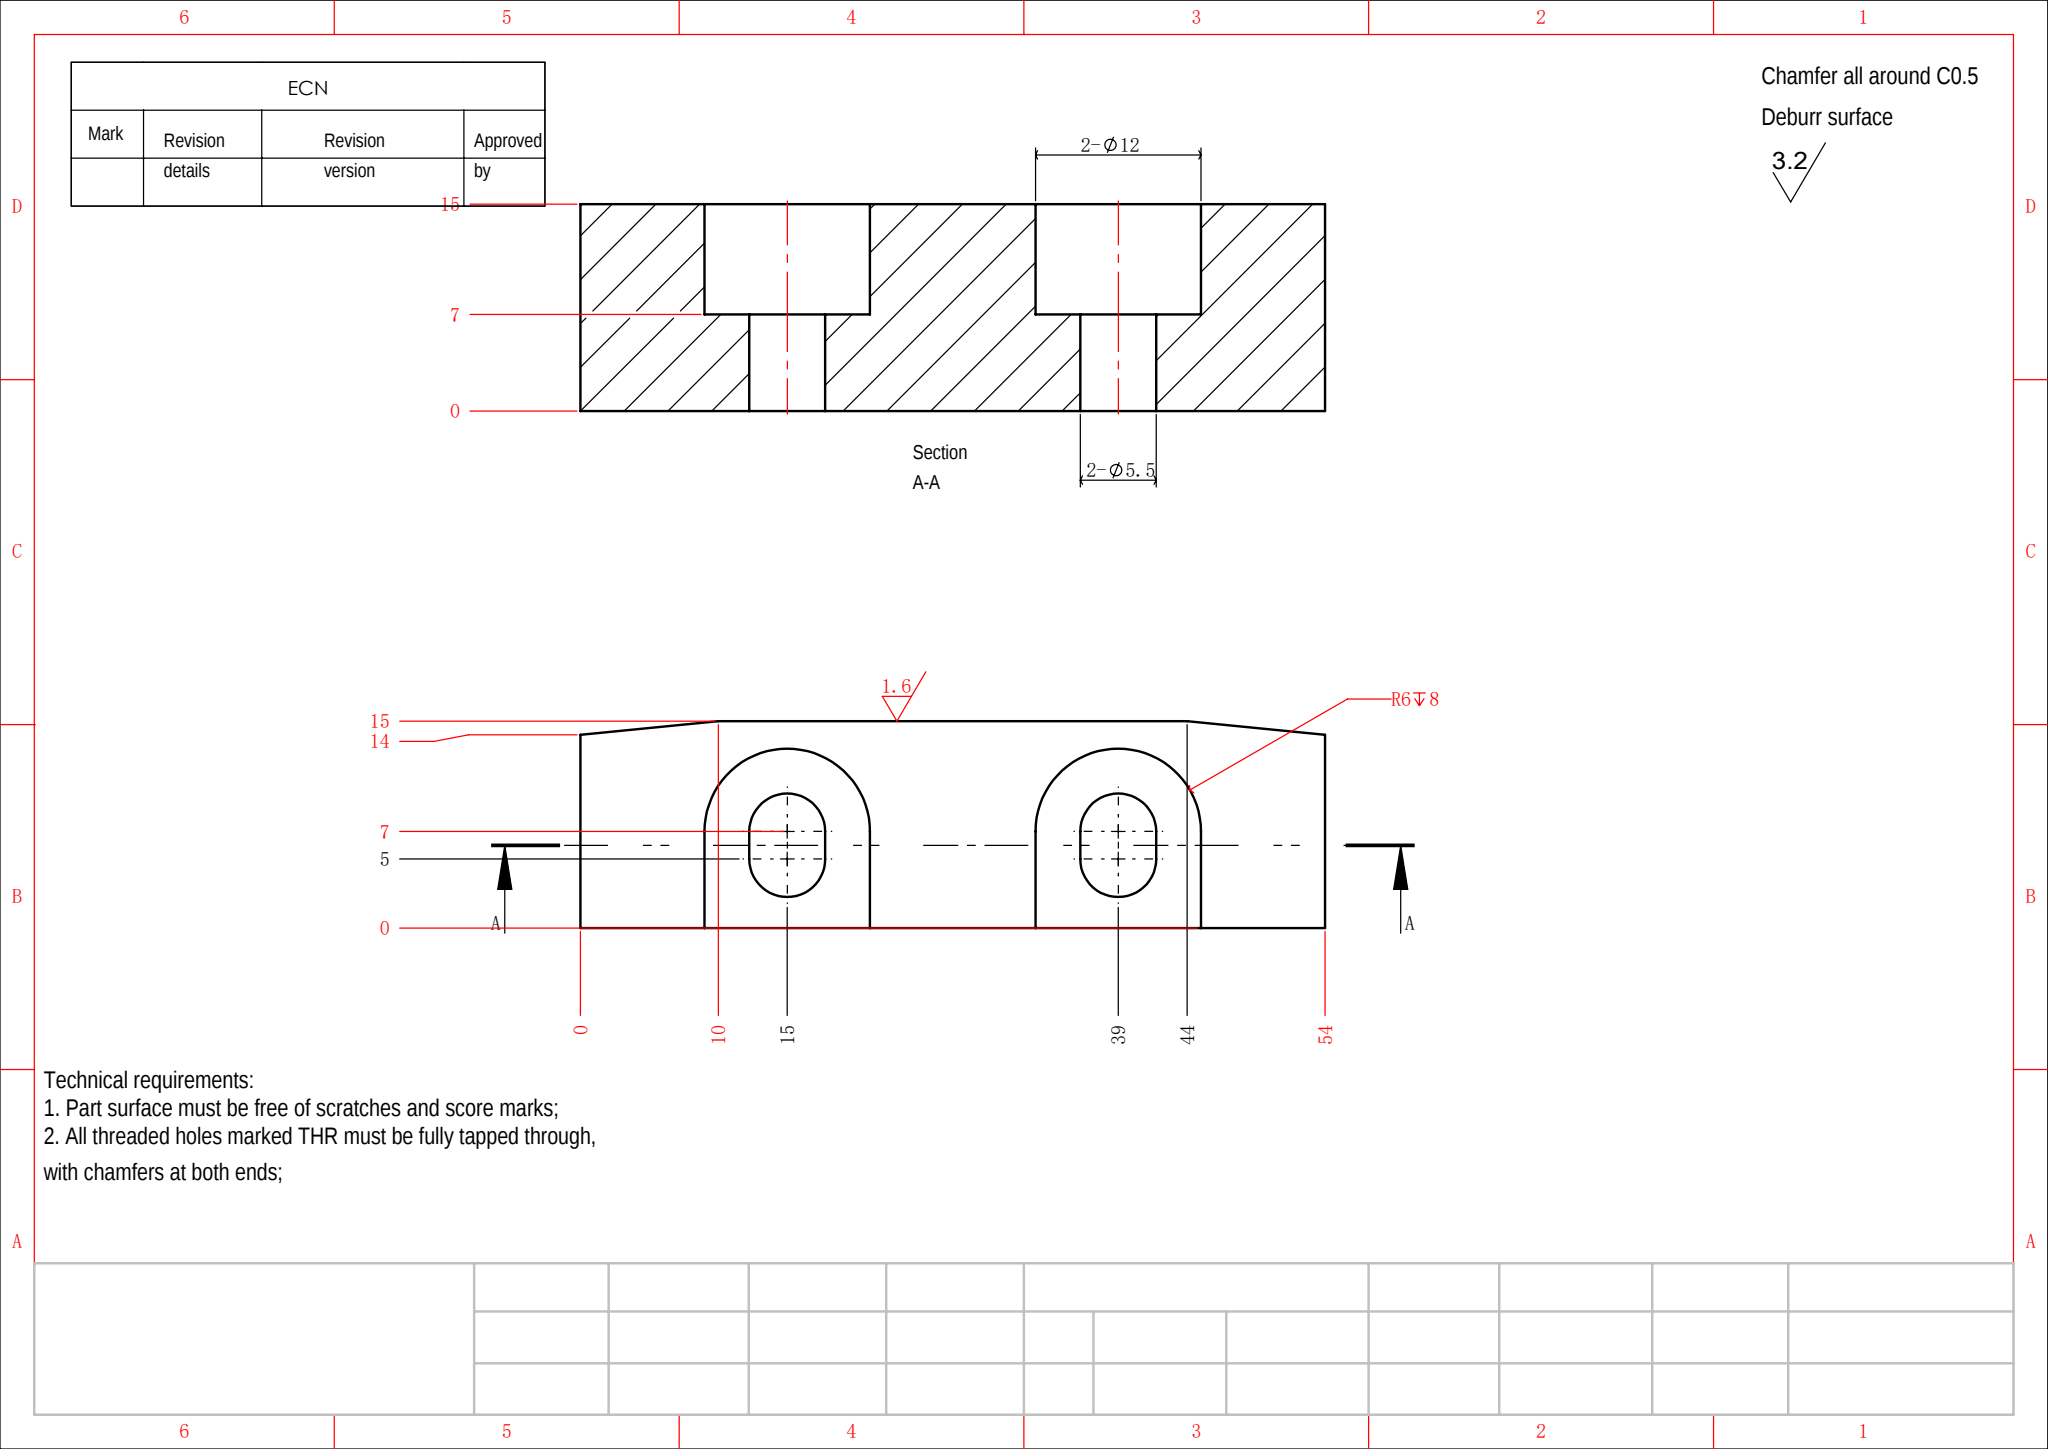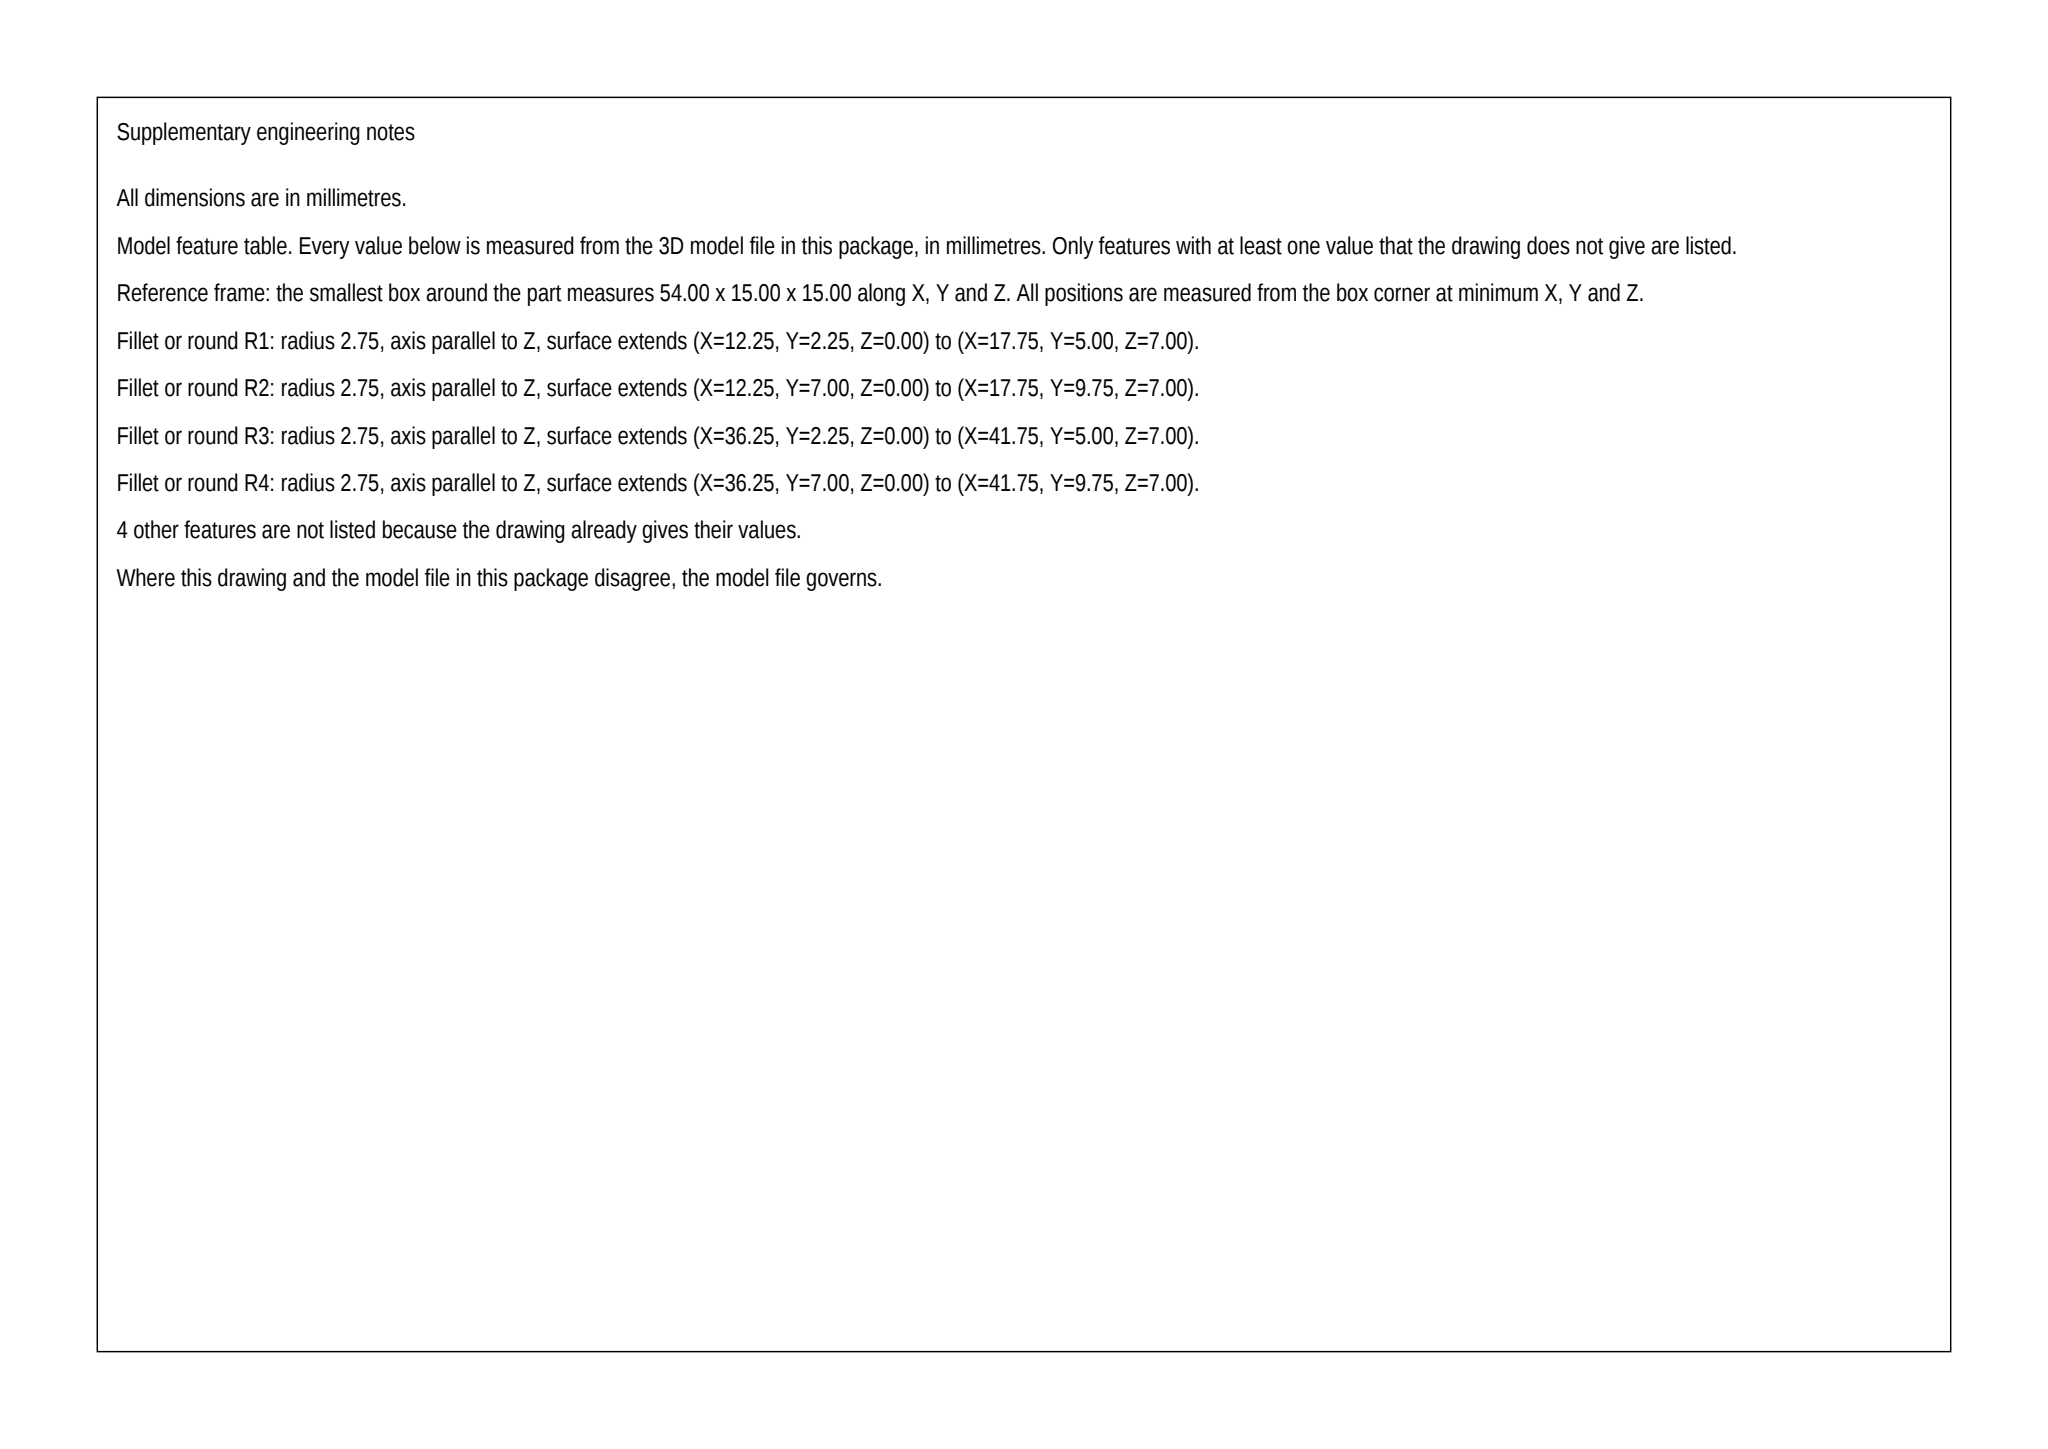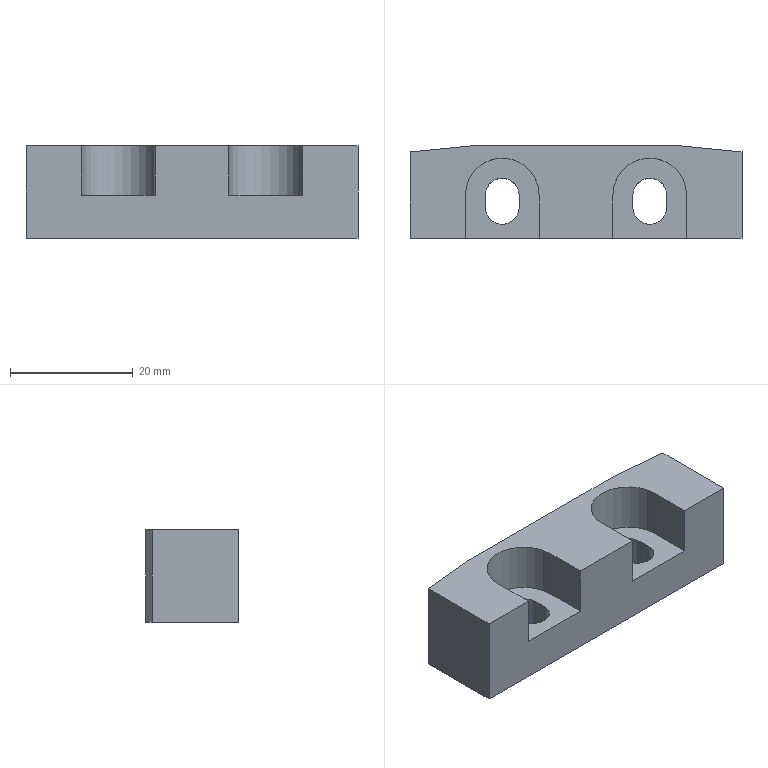Part | SolidWorks | mm | 1 solid | 24 faces | box 54 x 15 x 15 mm | volume 9265 mm3 | plane 18 | cylinder 6 | commonest cylinder face diameters 5.5 x4 12 x2
Drawing notes:
SECTION A-A: OVERALL HT 15 FROM BTM FACE (0 DATUM) | from the solid: z planes at 0.0 and 15.0; bbox_xyz z = 15.0
STEP:
#1=CARTESIAN_POINT('',(36.25,7.,0.));
#2=VERTEX_POINT('',#1);
#3=CARTESIAN_POINT('',(36.25,9.,0.));
#4=VERTEX_POINT('',#3);
#5=CARTESIAN_POINT('',(36.25,8.5,0.));
#6=DIRECTION('',(0.,1.,0.));
#7=VECTOR('',#6,1000.);
#8=LINE('',#5,#7);
#9=EDGE_CURVE('',#2,#4,#8,.T.);
#10=ORIENTED_EDGE('',*,*,#9,.F.);
#11=CARTESIAN_POINT('',(41.75,7.,0.));
#12=VERTEX_POINT('',#11);
#13=CARTESIAN_POINT('',(39.,7.,0.));
#14=DIRECTION('',(0.,0.,-1.));
#15=DIRECTION('',(-1.,0.,0.));
#16=AXIS2_PLACEMENT_3D('',#13,#14,#15);
#17=CIRCLE('',#16,2.75);
#18=EDGE_CURVE('',#12,#2,#17,.T.);
#19=ORIENTED_EDGE('',*,*,#18,.F.);
#20=CARTESIAN_POINT('',(41.75,9.,0.));
#21=VERTEX_POINT('',#20);
#22=CARTESIAN_POINT('',(41.75,8.5,0.));
#23=DIRECTION('',(0.,-1.,0.));
#24=VECTOR('',#23,1000.);
#25=LINE('',#22,#24);
#26=EDGE_CURVE('',#21,#12,#25,.T.);
#27=ORIENTED_EDGE('',*,*,#26,.F.);
#28=CARTESIAN_POINT('',(39.,9.,0.));
#29=DIRECTION('',(0.,0.,-1.));
#30=DIRECTION('',(-1.,0.,0.));
#31=AXIS2_PLACEMENT_3D('',#28,#29,#30);
#32=CIRCLE('',#31,2.75);
#33=EDGE_CURVE('',#4,#21,#32,.T.);
#34=ORIENTED_EDGE('',*,*,#33,.F.);
#35=EDGE_LOOP('',(#10,#19,#27,#34));
#36=FACE_BOUND('',#35,.T.);
#37=CARTESIAN_POINT('',(12.25,7.,0.));
#38=VERTEX_POINT('',#37);
#39=CARTESIAN_POINT('',(12.25,9.,0.));
#40=VERTEX_POINT('',#39);
#41=CARTESIAN_POINT('',(12.25,8.5,0.));
#42=DIRECTION('',(0.,1.,0.));
#43=VECTOR('',#42,1000.);
#44=LINE('',#41,#43);
#45=EDGE_CURVE('',#38,#40,#44,.T.);
#46=ORIENTED_EDGE('',*,*,#45,.F.);
#47=CARTESIAN_POINT('',(17.75,7.,0.));
#48=VERTEX_POINT('',#47);
#49=CARTESIAN_POINT('',(15.,7.,0.));
#50=DIRECTION('',(0.,0.,-1.));
#51=DIRECTION('',(-1.,0.,0.));
#52=AXIS2_PLACEMENT_3D('',#49,#50,#51);
#53=CIRCLE('',#52,2.75);
#54=EDGE_CURVE('',#48,#38,#53,.T.);
#55=ORIENTED_EDGE('',*,*,#54,.F.);
#56=CARTESIAN_POINT('',(17.75,9.,0.));
#57=VERTEX_POINT('',#56);
#58=CARTESIAN_POINT('',(17.75,8.5,0.));
#59=DIRECTION('',(0.,-1.,0.));
#60=VECTOR('',#59,1000.);
#61=LINE('',#58,#60);
#62=EDGE_CURVE('',#57,#48,#61,.T.);
#63=ORIENTED_EDGE('',*,*,#62,.F.);
#64=CARTESIAN_POINT('',(15.,9.,0.));
#65=DIRECTION('',(0.,0.,-1.));
#66=DIRECTION('',(-1.,0.,0.));
#67=AXIS2_PLACEMENT_3D('',#64,#65,#66);
#68=CIRCLE('',#67,2.75);
#69=EDGE_CURVE('',#40,#57,#68,.T.);
#70=ORIENTED_EDGE('',*,*,#69,.F.);
#71=EDGE_LOOP('',(#46,#55,#63,#70));
#72=FACE_BOUND('',#71,.T.);
#73=CARTESIAN_POINT('',(54.,2.,0.));
#74=VERTEX_POINT('',#73);
#75=CARTESIAN_POINT('',(54.,16.,0.));
#76=VERTEX_POINT('',#75);
#77=CARTESIAN_POINT('',(54.,8.5,0.));
#78=DIRECTION('',(0.,1.,0.));
#79=VECTOR('',#78,1000.);
#80=LINE('',#77,#79);
#81=EDGE_CURVE('',#74,#76,#80,.T.);
#82=ORIENTED_EDGE('',*,*,#81,.F.);
#83=CARTESIAN_POINT('',(-0.,2.,0.));
#84=VERTEX_POINT('',#83);
#85=CARTESIAN_POINT('',(27.,2.,0.));
#86=DIRECTION('',(1.,0.,0.));
#87=VECTOR('',#86,1000.);
#88=LINE('',#85,#87);
#89=EDGE_CURVE('',#84,#74,#88,.T.);
#90=ORIENTED_EDGE('',*,*,#89,.F.);
#91=CARTESIAN_POINT('',(-0.,16.,0.));
#92=VERTEX_POINT('',#91);
#93=CARTESIAN_POINT('',(-0.,8.5,0.));
#94=DIRECTION('',(0.,-1.,0.));
#95=VECTOR('',#94,1000.);
#96=LINE('',#93,#95);
#97=EDGE_CURVE('',#92,#84,#96,.T.);
#98=ORIENTED_EDGE('',*,*,#97,.F.);
#99=CARTESIAN_POINT('',(10.,17.,-0.));
#100=VERTEX_POINT('',#99);
#101=CARTESIAN_POINT('',(10.,17.,0.));
#102=DIRECTION('',(-0.995,-0.0995,0.));
#103=VECTOR('',#102,1000.);
#104=LINE('',#101,#103);
#105=EDGE_CURVE('',#100,#92,#104,.T.);
#106=ORIENTED_EDGE('',*,*,#105,.F.);
#107=CARTESIAN_POINT('',(44.,17.,-0.));
#108=VERTEX_POINT('',#107);
#109=CARTESIAN_POINT('',(27.,17.,0.));
#110=DIRECTION('',(-1.,0.,0.));
#111=VECTOR('',#110,1000.);
#112=LINE('',#109,#111);
#113=EDGE_CURVE('',#108,#100,#112,.T.);
#114=ORIENTED_EDGE('',*,*,#113,.F.);
#115=CARTESIAN_POINT('',(54.,16.,0.));
#116=DIRECTION('',(-0.995,0.0995,0.));
#117=VECTOR('',#116,1000.);
#118=LINE('',#115,#117);
#119=EDGE_CURVE('',#76,#108,#118,.T.);
#120=ORIENTED_EDGE('',*,*,#119,.F.);
#121=EDGE_LOOP('',(#82,#90,#98,#106,#114,#120));
#122=FACE_OUTER_BOUND('',#121,.T.);
#123=CARTESIAN_POINT('',(27.,8.5,0.));
#124=DIRECTION('',(0.,0.,1.));
#125=DIRECTION('',(1.,0.,0.));
#126=AXIS2_PLACEMENT_3D('',#123,#124,#125);
#127=PLANE('',#126);
#128=ADVANCED_FACE('',(#36,#72,#122),#127,.F.);
#129=CARTESIAN_POINT('',(36.25,9.,7.));
#130=VERTEX_POINT('',#129);
#131=CARTESIAN_POINT('',(36.25,9.,15.));
#132=DIRECTION('',(0.,0.,1.));
#133=VECTOR('',#132,1000.);
#134=LINE('',#131,#133);
#135=EDGE_CURVE('',#4,#130,#134,.T.);
#136=ORIENTED_EDGE('',*,*,#135,.F.);
#137=ORIENTED_EDGE('',*,*,#33,.T.);
#138=CARTESIAN_POINT('',(41.75,9.,7.));
#139=VERTEX_POINT('',#138);
#140=CARTESIAN_POINT('',(41.75,9.,15.));
#141=DIRECTION('',(0.,0.,-1.));
#142=VECTOR('',#141,1000.);
#143=LINE('',#140,#142);
#144=EDGE_CURVE('',#139,#21,#143,.T.);
#145=ORIENTED_EDGE('',*,*,#144,.F.);
#146=CARTESIAN_POINT('',(39.,9.,7.));
#147=DIRECTION('',(0.,0.,-1.));
#148=DIRECTION('',(-1.,0.,0.));
#149=AXIS2_PLACEMENT_3D('',#146,#147,#148);
#150=CIRCLE('',#149,2.75);
#151=EDGE_CURVE('',#130,#139,#150,.T.);
#152=ORIENTED_EDGE('',*,*,#151,.F.);
#153=EDGE_LOOP('',(#136,#137,#145,#152));
#154=FACE_OUTER_BOUND('',#153,.T.);
#155=CARTESIAN_POINT('',(39.,9.,15.));
#156=DIRECTION('',(0.,0.,-1.));
#157=DIRECTION('',(-1.,0.,0.));
#158=AXIS2_PLACEMENT_3D('',#155,#156,#157);
#159=CYLINDRICAL_SURFACE('',#158,2.75);
#160=ADVANCED_FACE('',(#154),#159,.F.);
#161=CARTESIAN_POINT('',(36.25,7.,7.));
#162=VERTEX_POINT('',#161);
#163=CARTESIAN_POINT('',(36.25,7.,15.));
#164=DIRECTION('',(0.,0.,1.));
#165=VECTOR('',#164,1000.);
#166=LINE('',#163,#165);
#167=EDGE_CURVE('',#2,#162,#166,.T.);
#168=ORIENTED_EDGE('',*,*,#167,.F.);
#169=ORIENTED_EDGE('',*,*,#9,.T.);
#170=ORIENTED_EDGE('',*,*,#135,.T.);
#171=CARTESIAN_POINT('',(36.25,7.,7.));
#172=DIRECTION('',(0.,1.,0.));
#173=VECTOR('',#172,1000.);
#174=LINE('',#171,#173);
#175=EDGE_CURVE('',#162,#130,#174,.T.);
#176=ORIENTED_EDGE('',*,*,#175,.F.);
#177=EDGE_LOOP('',(#168,#169,#170,#176));
#178=FACE_OUTER_BOUND('',#177,.T.);
#179=CARTESIAN_POINT('',(36.25,7.,15.));
#180=DIRECTION('',(-1.,0.,0.));
#181=DIRECTION('',(0.,0.,1.));
#182=AXIS2_PLACEMENT_3D('',#179,#180,#181);
#183=PLANE('',#182);
#184=ADVANCED_FACE('',(#178),#183,.F.);
#185=CARTESIAN_POINT('',(41.75,7.,7.));
#186=VERTEX_POINT('',#185);
#187=CARTESIAN_POINT('',(41.75,7.,15.));
#188=DIRECTION('',(0.,0.,1.));
#189=VECTOR('',#188,1000.);
#190=LINE('',#187,#189);
#191=EDGE_CURVE('',#12,#186,#190,.T.);
#192=ORIENTED_EDGE('',*,*,#191,.F.);
#193=ORIENTED_EDGE('',*,*,#18,.T.);
#194=ORIENTED_EDGE('',*,*,#167,.T.);
#195=CARTESIAN_POINT('',(39.,7.,7.));
#196=DIRECTION('',(0.,0.,-1.));
#197=DIRECTION('',(-1.,0.,0.));
#198=AXIS2_PLACEMENT_3D('',#195,#196,#197);
#199=CIRCLE('',#198,2.75);
#200=EDGE_CURVE('',#186,#162,#199,.T.);
#201=ORIENTED_EDGE('',*,*,#200,.F.);
#202=EDGE_LOOP('',(#192,#193,#194,#201));
#203=FACE_OUTER_BOUND('',#202,.T.);
#204=CARTESIAN_POINT('',(39.,7.,15.));
#205=DIRECTION('',(0.,0.,-1.));
#206=DIRECTION('',(-1.,0.,0.));
#207=AXIS2_PLACEMENT_3D('',#204,#205,#206);
#208=CYLINDRICAL_SURFACE('',#207,2.75);
#209=ADVANCED_FACE('',(#203),#208,.F.);
#210=ORIENTED_EDGE('',*,*,#144,.T.);
#211=ORIENTED_EDGE('',*,*,#26,.T.);
#212=ORIENTED_EDGE('',*,*,#191,.T.);
#213=CARTESIAN_POINT('',(41.75,9.,7.));
#214=DIRECTION('',(-0.,-1.,0.));
#215=VECTOR('',#214,1000.);
#216=LINE('',#213,#215);
#217=EDGE_CURVE('',#139,#186,#216,.T.);
#218=ORIENTED_EDGE('',*,*,#217,.F.);
#219=EDGE_LOOP('',(#210,#211,#212,#218));
#220=FACE_OUTER_BOUND('',#219,.T.);
#221=CARTESIAN_POINT('',(41.75,9.,15.));
#222=DIRECTION('',(1.,-0.,0.));
#223=DIRECTION('',(0.,1.,0.));
#224=AXIS2_PLACEMENT_3D('',#221,#222,#223);
#225=PLANE('',#224);
#226=ADVANCED_FACE('',(#220),#225,.F.);
#227=CARTESIAN_POINT('',(12.25,9.,7.));
#228=VERTEX_POINT('',#227);
#229=CARTESIAN_POINT('',(12.25,9.,15.));
#230=DIRECTION('',(0.,0.,1.));
#231=VECTOR('',#230,1000.);
#232=LINE('',#229,#231);
#233=EDGE_CURVE('',#40,#228,#232,.T.);
#234=ORIENTED_EDGE('',*,*,#233,.F.);
#235=ORIENTED_EDGE('',*,*,#69,.T.);
#236=CARTESIAN_POINT('',(17.75,9.,7.));
#237=VERTEX_POINT('',#236);
#238=CARTESIAN_POINT('',(17.75,9.,15.));
#239=DIRECTION('',(0.,0.,-1.));
#240=VECTOR('',#239,1000.);
#241=LINE('',#238,#240);
#242=EDGE_CURVE('',#237,#57,#241,.T.);
#243=ORIENTED_EDGE('',*,*,#242,.F.);
#244=CARTESIAN_POINT('',(15.,9.,7.));
#245=DIRECTION('',(0.,0.,-1.));
#246=DIRECTION('',(-1.,0.,0.));
#247=AXIS2_PLACEMENT_3D('',#244,#245,#246);
#248=CIRCLE('',#247,2.75);
#249=EDGE_CURVE('',#228,#237,#248,.T.);
#250=ORIENTED_EDGE('',*,*,#249,.F.);
#251=EDGE_LOOP('',(#234,#235,#243,#250));
#252=FACE_OUTER_BOUND('',#251,.T.);
#253=CARTESIAN_POINT('',(15.,9.,15.));
#254=DIRECTION('',(0.,0.,-1.));
#255=DIRECTION('',(-1.,0.,0.));
#256=AXIS2_PLACEMENT_3D('',#253,#254,#255);
#257=CYLINDRICAL_SURFACE('',#256,2.75);
#258=ADVANCED_FACE('',(#252),#257,.F.);
#259=CARTESIAN_POINT('',(12.25,7.,7.));
#260=VERTEX_POINT('',#259);
#261=CARTESIAN_POINT('',(12.25,7.,15.));
#262=DIRECTION('',(0.,0.,1.));
#263=VECTOR('',#262,1000.);
#264=LINE('',#261,#263);
#265=EDGE_CURVE('',#38,#260,#264,.T.);
#266=ORIENTED_EDGE('',*,*,#265,.F.);
#267=ORIENTED_EDGE('',*,*,#45,.T.);
#268=ORIENTED_EDGE('',*,*,#233,.T.);
#269=CARTESIAN_POINT('',(12.25,7.,7.));
#270=DIRECTION('',(-0.,1.,0.));
#271=VECTOR('',#270,1000.);
#272=LINE('',#269,#271);
#273=EDGE_CURVE('',#260,#228,#272,.T.);
#274=ORIENTED_EDGE('',*,*,#273,.F.);
#275=EDGE_LOOP('',(#266,#267,#268,#274));
#276=FACE_OUTER_BOUND('',#275,.T.);
#277=CARTESIAN_POINT('',(12.25,7.,15.));
#278=DIRECTION('',(-1.,-0.,0.));
#279=DIRECTION('',(0.,-1.,0.));
#280=AXIS2_PLACEMENT_3D('',#277,#278,#279);
#281=PLANE('',#280);
#282=ADVANCED_FACE('',(#276),#281,.F.);
#283=CARTESIAN_POINT('',(17.75,7.,7.));
#284=VERTEX_POINT('',#283);
#285=CARTESIAN_POINT('',(17.75,7.,15.));
#286=DIRECTION('',(0.,0.,1.));
#287=VECTOR('',#286,1000.);
#288=LINE('',#285,#287);
#289=EDGE_CURVE('',#48,#284,#288,.T.);
#290=ORIENTED_EDGE('',*,*,#289,.F.);
#291=ORIENTED_EDGE('',*,*,#54,.T.);
#292=ORIENTED_EDGE('',*,*,#265,.T.);
#293=CARTESIAN_POINT('',(15.,7.,7.));
#294=DIRECTION('',(0.,0.,-1.));
#295=DIRECTION('',(-1.,0.,0.));
#296=AXIS2_PLACEMENT_3D('',#293,#294,#295);
#297=CIRCLE('',#296,2.75);
#298=EDGE_CURVE('',#284,#260,#297,.T.);
#299=ORIENTED_EDGE('',*,*,#298,.F.);
#300=EDGE_LOOP('',(#290,#291,#292,#299));
#301=FACE_OUTER_BOUND('',#300,.T.);
#302=CARTESIAN_POINT('',(15.,7.,15.));
#303=DIRECTION('',(0.,0.,-1.));
#304=DIRECTION('',(-1.,0.,0.));
#305=AXIS2_PLACEMENT_3D('',#302,#303,#304);
#306=CYLINDRICAL_SURFACE('',#305,2.75);
#307=ADVANCED_FACE('',(#301),#306,.F.);
#308=ORIENTED_EDGE('',*,*,#242,.T.);
#309=ORIENTED_EDGE('',*,*,#62,.T.);
#310=ORIENTED_EDGE('',*,*,#289,.T.);
#311=CARTESIAN_POINT('',(17.75,9.,7.));
#312=DIRECTION('',(0.,-1.,0.));
#313=VECTOR('',#312,1000.);
#314=LINE('',#311,#313);
#315=EDGE_CURVE('',#237,#284,#314,.T.);
#316=ORIENTED_EDGE('',*,*,#315,.F.);
#317=EDGE_LOOP('',(#308,#309,#310,#316));
#318=FACE_OUTER_BOUND('',#317,.T.);
#319=CARTESIAN_POINT('',(17.75,9.,15.));
#320=DIRECTION('',(1.,0.,0.));
#321=DIRECTION('',(0.,0.,-1.));
#322=AXIS2_PLACEMENT_3D('',#319,#320,#321);
#323=PLANE('',#322);
#324=ADVANCED_FACE('',(#318),#323,.F.);
#325=ORIENTED_EDGE('',*,*,#119,.T.);
#326=CARTESIAN_POINT('',(44.,17.,15.));
#327=VERTEX_POINT('',#326);
#328=CARTESIAN_POINT('',(44.,17.,0.));
#329=DIRECTION('',(0.,0.,1.));
#330=VECTOR('',#329,1000.);
#331=LINE('',#328,#330);
#332=EDGE_CURVE('',#108,#327,#331,.T.);
#333=ORIENTED_EDGE('',*,*,#332,.T.);
#334=CARTESIAN_POINT('',(54.,16.,15.));
#335=VERTEX_POINT('',#334);
#336=CARTESIAN_POINT('',(49.,16.5,15.));
#337=DIRECTION('',(0.995,-0.0995,0.));
#338=VECTOR('',#337,1000.);
#339=LINE('',#336,#338);
#340=EDGE_CURVE('',#327,#335,#339,.T.);
#341=ORIENTED_EDGE('',*,*,#340,.T.);
#342=CARTESIAN_POINT('',(54.,16.,0.));
#343=DIRECTION('',(0.,0.,-1.));
#344=VECTOR('',#343,1000.);
#345=LINE('',#342,#344);
#346=EDGE_CURVE('',#335,#76,#345,.T.);
#347=ORIENTED_EDGE('',*,*,#346,.T.);
#348=EDGE_LOOP('',(#325,#333,#341,#347));
#349=FACE_OUTER_BOUND('',#348,.T.);
#350=CARTESIAN_POINT('',(49.,16.5,0.));
#351=DIRECTION('',(0.0995,0.995,0.));
#352=DIRECTION('',(-0.995,0.0995,0.));
#353=AXIS2_PLACEMENT_3D('',#350,#351,#352);
#354=PLANE('',#353);
#355=ADVANCED_FACE('',(#349),#354,.T.);
#356=CARTESIAN_POINT('',(54.,2.,15.));
#357=VERTEX_POINT('',#356);
#358=CARTESIAN_POINT('',(54.,2.,0.));
#359=DIRECTION('',(0.,0.,-1.));
#360=VECTOR('',#359,1000.);
#361=LINE('',#358,#360);
#362=EDGE_CURVE('',#357,#74,#361,.T.);
#363=ORIENTED_EDGE('',*,*,#362,.T.);
#364=ORIENTED_EDGE('',*,*,#81,.T.);
#365=ORIENTED_EDGE('',*,*,#346,.F.);
#366=CARTESIAN_POINT('',(54.,-0.,15.));
#367=DIRECTION('',(0.,-1.,0.));
#368=VECTOR('',#367,1000.);
#369=LINE('',#366,#368);
#370=EDGE_CURVE('',#335,#357,#369,.T.);
#371=ORIENTED_EDGE('',*,*,#370,.T.);
#372=EDGE_LOOP('',(#363,#364,#365,#371));
#373=FACE_OUTER_BOUND('',#372,.T.);
#374=CARTESIAN_POINT('',(54.,-0.,0.));
#375=DIRECTION('',(1.,0.,0.));
#376=DIRECTION('',(0.,0.,-1.));
#377=AXIS2_PLACEMENT_3D('',#374,#375,#376);
#378=PLANE('',#377);
#379=ADVANCED_FACE('',(#373),#378,.T.);
#380=CARTESIAN_POINT('',(33.,2.,7.));
#381=VERTEX_POINT('',#380);
#382=CARTESIAN_POINT('',(33.,2.,15.));
#383=VERTEX_POINT('',#382);
#384=CARTESIAN_POINT('',(33.,2.,-6.892));
#385=DIRECTION('',(0.,0.,1.));
#386=VECTOR('',#385,1000.);
#387=LINE('',#384,#386);
#388=EDGE_CURVE('',#381,#383,#387,.T.);
#389=ORIENTED_EDGE('',*,*,#388,.T.);
#390=CARTESIAN_POINT('',(21.,2.,15.));
#391=VERTEX_POINT('',#390);
#392=CARTESIAN_POINT('',(0.,2.,15.));
#393=DIRECTION('',(-1.,0.,0.));
#394=VECTOR('',#393,1000.);
#395=LINE('',#392,#394);
#396=EDGE_CURVE('',#383,#391,#395,.T.);
#397=ORIENTED_EDGE('',*,*,#396,.T.);
#398=CARTESIAN_POINT('',(21.,2.,7.));
#399=VERTEX_POINT('',#398);
#400=CARTESIAN_POINT('',(21.,2.,-6.892));
#401=DIRECTION('',(0.,0.,1.));
#402=VECTOR('',#401,1000.);
#403=LINE('',#400,#402);
#404=EDGE_CURVE('',#399,#391,#403,.T.);
#405=ORIENTED_EDGE('',*,*,#404,.F.);
#406=CARTESIAN_POINT('',(9.,2.,7.));
#407=VERTEX_POINT('',#406);
#408=CARTESIAN_POINT('',(9.,2.,7.));
#409=DIRECTION('',(-1.,0.,0.));
#410=VECTOR('',#409,1000.);
#411=LINE('',#408,#410);
#412=EDGE_CURVE('',#399,#407,#411,.T.);
#413=ORIENTED_EDGE('',*,*,#412,.T.);
#414=CARTESIAN_POINT('',(9.,2.,15.));
#415=VERTEX_POINT('',#414);
#416=CARTESIAN_POINT('',(9.,2.,-6.892));
#417=DIRECTION('',(0.,0.,1.));
#418=VECTOR('',#417,1000.);
#419=LINE('',#416,#418);
#420=EDGE_CURVE('',#407,#415,#419,.T.);
#421=ORIENTED_EDGE('',*,*,#420,.T.);
#422=CARTESIAN_POINT('',(-0.,2.,15.));
#423=VERTEX_POINT('',#422);
#424=CARTESIAN_POINT('',(0.,2.,15.));
#425=DIRECTION('',(-1.,0.,0.));
#426=VECTOR('',#425,1000.);
#427=LINE('',#424,#426);
#428=EDGE_CURVE('',#415,#423,#427,.T.);
#429=ORIENTED_EDGE('',*,*,#428,.T.);
#430=CARTESIAN_POINT('',(0.,2.,0.));
#431=DIRECTION('',(0.,0.,-1.));
#432=VECTOR('',#431,1000.);
#433=LINE('',#430,#432);
#434=EDGE_CURVE('',#423,#84,#433,.T.);
#435=ORIENTED_EDGE('',*,*,#434,.T.);
#436=ORIENTED_EDGE('',*,*,#89,.T.);
#437=ORIENTED_EDGE('',*,*,#362,.F.);
#438=CARTESIAN_POINT('',(45.,2.,15.));
#439=VERTEX_POINT('',#438);
#440=CARTESIAN_POINT('',(0.,2.,15.));
#441=DIRECTION('',(-1.,0.,0.));
#442=VECTOR('',#441,1000.);
#443=LINE('',#440,#442);
#444=EDGE_CURVE('',#357,#439,#443,.T.);
#445=ORIENTED_EDGE('',*,*,#444,.T.);
#446=CARTESIAN_POINT('',(45.,2.,7.));
#447=VERTEX_POINT('',#446);
#448=CARTESIAN_POINT('',(45.,2.,-6.892));
#449=DIRECTION('',(0.,0.,1.));
#450=VECTOR('',#449,1000.);
#451=LINE('',#448,#450);
#452=EDGE_CURVE('',#447,#439,#451,.T.);
#453=ORIENTED_EDGE('',*,*,#452,.F.);
#454=CARTESIAN_POINT('',(33.,2.,7.));
#455=DIRECTION('',(-1.,0.,0.));
#456=VECTOR('',#455,1000.);
#457=LINE('',#454,#456);
#458=EDGE_CURVE('',#447,#381,#457,.T.);
#459=ORIENTED_EDGE('',*,*,#458,.T.);
#460=EDGE_LOOP('',(#389,#397,#405,#413,#421,#429,#435,#436,#437,#445,#453,#459));
#461=FACE_OUTER_BOUND('',#460,.T.);
#462=CARTESIAN_POINT('',(0.,2.,0.));
#463=DIRECTION('',(-0.,-1.,0.));
#464=DIRECTION('',(1.,-0.,0.));
#465=AXIS2_PLACEMENT_3D('',#462,#463,#464);
#466=PLANE('',#465);
#467=ADVANCED_FACE('',(#461),#466,.T.);
#468=ORIENTED_EDGE('',*,*,#434,.F.);
#469=CARTESIAN_POINT('',(-0.,16.,15.));
#470=VERTEX_POINT('',#469);
#471=CARTESIAN_POINT('',(-0.,17.,15.));
#472=DIRECTION('',(-0.,1.,0.));
#473=VECTOR('',#472,1000.);
#474=LINE('',#471,#473);
#475=EDGE_CURVE('',#423,#470,#474,.T.);
#476=ORIENTED_EDGE('',*,*,#475,.T.);
#477=CARTESIAN_POINT('',(-0.,16.,0.));
#478=DIRECTION('',(0.,0.,-1.));
#479=VECTOR('',#478,1000.);
#480=LINE('',#477,#479);
#481=EDGE_CURVE('',#470,#92,#480,.T.);
#482=ORIENTED_EDGE('',*,*,#481,.T.);
#483=ORIENTED_EDGE('',*,*,#97,.T.);
#484=EDGE_LOOP('',(#468,#476,#482,#483));
#485=FACE_OUTER_BOUND('',#484,.T.);
#486=CARTESIAN_POINT('',(-0.,17.,0.));
#487=DIRECTION('',(-1.,-0.,0.));
#488=DIRECTION('',(0.,-1.,0.));
#489=AXIS2_PLACEMENT_3D('',#486,#487,#488);
#490=PLANE('',#489);
#491=ADVANCED_FACE('',(#485),#490,.T.);
#492=ORIENTED_EDGE('',*,*,#105,.T.);
#493=ORIENTED_EDGE('',*,*,#481,.F.);
#494=CARTESIAN_POINT('',(10.,17.,15.));
#495=VERTEX_POINT('',#494);
#496=CARTESIAN_POINT('',(5.,16.5,15.));
#497=DIRECTION('',(0.995,0.0995,0.));
#498=VECTOR('',#497,1000.);
#499=LINE('',#496,#498);
#500=EDGE_CURVE('',#470,#495,#499,.T.);
#501=ORIENTED_EDGE('',*,*,#500,.T.);
#502=CARTESIAN_POINT('',(10.,17.,0.));
#503=DIRECTION('',(0.,0.,-1.));
#504=VECTOR('',#503,1000.);
#505=LINE('',#502,#504);
#506=EDGE_CURVE('',#495,#100,#505,.T.);
#507=ORIENTED_EDGE('',*,*,#506,.T.);
#508=EDGE_LOOP('',(#492,#493,#501,#507));
#509=FACE_OUTER_BOUND('',#508,.T.);
#510=CARTESIAN_POINT('',(5.,16.5,0.));
#511=DIRECTION('',(-0.0995,0.995,0.));
#512=DIRECTION('',(-0.995,-0.0995,0.));
#513=AXIS2_PLACEMENT_3D('',#510,#511,#512);
#514=PLANE('',#513);
#515=ADVANCED_FACE('',(#509),#514,.T.);
#516=ORIENTED_EDGE('',*,*,#506,.F.);
#517=CARTESIAN_POINT('',(54.,17.,15.));
#518=DIRECTION('',(1.,0.,0.));
#519=VECTOR('',#518,1000.);
#520=LINE('',#517,#519);
#521=EDGE_CURVE('',#495,#327,#520,.T.);
#522=ORIENTED_EDGE('',*,*,#521,.T.);
#523=ORIENTED_EDGE('',*,*,#332,.F.);
#524=ORIENTED_EDGE('',*,*,#113,.T.);
#525=EDGE_LOOP('',(#516,#522,#523,#524));
#526=FACE_OUTER_BOUND('',#525,.T.);
#527=CARTESIAN_POINT('',(54.,17.,0.));
#528=DIRECTION('',(-0.,1.,0.));
#529=DIRECTION('',(0.,-0.,1.));
#530=AXIS2_PLACEMENT_3D('',#527,#528,#529);
#531=PLANE('',#530);
#532=ADVANCED_FACE('',(#526),#531,.T.);
#533=ORIENTED_EDGE('',*,*,#217,.T.);
#534=ORIENTED_EDGE('',*,*,#200,.T.);
#535=ORIENTED_EDGE('',*,*,#175,.T.);
#536=ORIENTED_EDGE('',*,*,#151,.T.);
#537=EDGE_LOOP('',(#533,#534,#535,#536));
#538=FACE_BOUND('',#537,.T.);
#539=CARTESIAN_POINT('',(33.,9.,7.));
#540=VERTEX_POINT('',#539);
#541=CARTESIAN_POINT('',(33.,8.,7.));
#542=DIRECTION('',(0.,-1.,0.));
#543=VECTOR('',#542,1000.);
#544=LINE('',#541,#543);
#545=EDGE_CURVE('',#540,#381,#544,.T.);
#546=ORIENTED_EDGE('',*,*,#545,.T.);
#547=ORIENTED_EDGE('',*,*,#458,.F.);
#548=CARTESIAN_POINT('',(45.,9.,7.));
#549=VERTEX_POINT('',#548);
#550=CARTESIAN_POINT('',(45.,8.,7.));
#551=DIRECTION('',(0.,1.,0.));
#552=VECTOR('',#551,1000.);
#553=LINE('',#550,#552);
#554=EDGE_CURVE('',#447,#549,#553,.T.);
#555=ORIENTED_EDGE('',*,*,#554,.T.);
#556=CARTESIAN_POINT('',(39.,9.,7.));
#557=DIRECTION('',(0.,0.,1.));
#558=DIRECTION('',(-1.,0.,0.));
#559=AXIS2_PLACEMENT_3D('',#556,#557,#558);
#560=CIRCLE('',#559,6.);
#561=EDGE_CURVE('',#549,#540,#560,.T.);
#562=ORIENTED_EDGE('',*,*,#561,.T.);
#563=EDGE_LOOP('',(#546,#547,#555,#562));
#564=FACE_OUTER_BOUND('',#563,.T.);
#565=CARTESIAN_POINT('',(39.,8.,7.));
#566=DIRECTION('',(0.,0.,1.));
#567=DIRECTION('',(1.,0.,0.));
#568=AXIS2_PLACEMENT_3D('',#565,#566,#567);
#569=PLANE('',#568);
#570=ADVANCED_FACE('',(#538,#564),#569,.T.);
#571=ORIENTED_EDGE('',*,*,#315,.T.);
#572=ORIENTED_EDGE('',*,*,#298,.T.);
#573=ORIENTED_EDGE('',*,*,#273,.T.);
#574=ORIENTED_EDGE('',*,*,#249,.T.);
#575=EDGE_LOOP('',(#571,#572,#573,#574));
#576=FACE_BOUND('',#575,.T.);
#577=CARTESIAN_POINT('',(9.,9.,7.));
#578=VERTEX_POINT('',#577);
#579=CARTESIAN_POINT('',(9.,8.,7.));
#580=DIRECTION('',(0.,-1.,0.));
#581=VECTOR('',#580,1000.);
#582=LINE('',#579,#581);
#583=EDGE_CURVE('',#578,#407,#582,.T.);
#584=ORIENTED_EDGE('',*,*,#583,.T.);
#585=ORIENTED_EDGE('',*,*,#412,.F.);
#586=CARTESIAN_POINT('',(21.,9.,7.));
#587=VERTEX_POINT('',#586);
#588=CARTESIAN_POINT('',(21.,8.,7.));
#589=DIRECTION('',(0.,1.,0.));
#590=VECTOR('',#589,1000.);
#591=LINE('',#588,#590);
#592=EDGE_CURVE('',#399,#587,#591,.T.);
#593=ORIENTED_EDGE('',*,*,#592,.T.);
#594=CARTESIAN_POINT('',(15.,9.,7.));
#595=DIRECTION('',(0.,0.,1.));
#596=DIRECTION('',(-1.,0.,0.));
#597=AXIS2_PLACEMENT_3D('',#594,#595,#596);
#598=CIRCLE('',#597,6.);
#599=EDGE_CURVE('',#587,#578,#598,.T.);
#600=ORIENTED_EDGE('',*,*,#599,.T.);
#601=EDGE_LOOP('',(#584,#585,#593,#600));
#602=FACE_OUTER_BOUND('',#601,.T.);
#603=CARTESIAN_POINT('',(15.,8.,7.));
#604=DIRECTION('',(0.,0.,1.));
#605=DIRECTION('',(1.,0.,0.));
#606=AXIS2_PLACEMENT_3D('',#603,#604,#605);
#607=PLANE('',#606);
#608=ADVANCED_FACE('',(#576,#602),#607,.T.);
#609=ORIENTED_EDGE('',*,*,#396,.F.);
#610=CARTESIAN_POINT('',(33.,9.,15.));
#611=VERTEX_POINT('',#610);
#612=CARTESIAN_POINT('',(33.,8.5,15.));
#613=DIRECTION('',(0.,1.,0.));
#614=VECTOR('',#613,1000.);
#615=LINE('',#612,#614);
#616=EDGE_CURVE('',#383,#611,#615,.T.);
#617=ORIENTED_EDGE('',*,*,#616,.T.);
#618=CARTESIAN_POINT('',(45.,9.,15.));
#619=VERTEX_POINT('',#618);
#620=CARTESIAN_POINT('',(39.,9.,15.));
#621=DIRECTION('',(0.,0.,-1.));
#622=DIRECTION('',(-1.,0.,0.));
#623=AXIS2_PLACEMENT_3D('',#620,#621,#622);
#624=CIRCLE('',#623,6.);
#625=EDGE_CURVE('',#611,#619,#624,.T.);
#626=ORIENTED_EDGE('',*,*,#625,.T.);
#627=CARTESIAN_POINT('',(45.,8.5,15.));
#628=DIRECTION('',(0.,-1.,0.));
#629=VECTOR('',#628,1000.);
#630=LINE('',#627,#629);
#631=EDGE_CURVE('',#619,#439,#630,.T.);
#632=ORIENTED_EDGE('',*,*,#631,.T.);
#633=ORIENTED_EDGE('',*,*,#444,.F.);
#634=ORIENTED_EDGE('',*,*,#370,.F.);
#635=ORIENTED_EDGE('',*,*,#340,.F.);
#636=ORIENTED_EDGE('',*,*,#521,.F.);
#637=ORIENTED_EDGE('',*,*,#500,.F.);
#638=ORIENTED_EDGE('',*,*,#475,.F.);
#639=ORIENTED_EDGE('',*,*,#428,.F.);
#640=CARTESIAN_POINT('',(9.,9.,15.));
#641=VERTEX_POINT('',#640);
#642=CARTESIAN_POINT('',(9.,8.5,15.));
#643=DIRECTION('',(0.,1.,0.));
#644=VECTOR('',#643,1000.);
#645=LINE('',#642,#644);
#646=EDGE_CURVE('',#415,#641,#645,.T.);
#647=ORIENTED_EDGE('',*,*,#646,.T.);
#648=CARTESIAN_POINT('',(21.,9.,15.));
#649=VERTEX_POINT('',#648);
#650=CARTESIAN_POINT('',(15.,9.,15.));
#651=DIRECTION('',(0.,0.,-1.));
#652=DIRECTION('',(-1.,0.,0.));
#653=AXIS2_PLACEMENT_3D('',#650,#651,#652);
#654=CIRCLE('',#653,6.);
#655=EDGE_CURVE('',#641,#649,#654,.T.);
#656=ORIENTED_EDGE('',*,*,#655,.T.);
#657=CARTESIAN_POINT('',(21.,8.5,15.));
#658=DIRECTION('',(0.,-1.,0.));
#659=VECTOR('',#658,1000.);
#660=LINE('',#657,#659);
#661=EDGE_CURVE('',#649,#391,#660,.T.);
#662=ORIENTED_EDGE('',*,*,#661,.T.);
#663=EDGE_LOOP('',(#609,#617,#626,#632,#633,#634,#635,#636,#637,#638,#639,#647,#656,#662));
#664=FACE_OUTER_BOUND('',#663,.T.);
#665=CARTESIAN_POINT('',(27.,8.5,15.));
#666=DIRECTION('',(0.,0.,1.));
#667=DIRECTION('',(1.,0.,0.));
#668=AXIS2_PLACEMENT_3D('',#665,#666,#667);
#669=PLANE('',#668);
#670=ADVANCED_FACE('',(#664),#669,.T.);
#671=CARTESIAN_POINT('',(33.,9.,15.));
#672=DIRECTION('',(0.,0.,1.));
#673=VECTOR('',#672,1000.);
#674=LINE('',#671,#673);
#675=EDGE_CURVE('',#540,#611,#674,.T.);
#676=ORIENTED_EDGE('',*,*,#675,.F.);
#677=ORIENTED_EDGE('',*,*,#561,.F.);
#678=CARTESIAN_POINT('',(45.,9.,15.));
#679=DIRECTION('',(0.,0.,-1.));
#680=VECTOR('',#679,1000.);
#681=LINE('',#678,#680);
#682=EDGE_CURVE('',#619,#549,#681,.T.);
#683=ORIENTED_EDGE('',*,*,#682,.F.);
#684=ORIENTED_EDGE('',*,*,#625,.F.);
#685=EDGE_LOOP('',(#676,#677,#683,#684));
#686=FACE_OUTER_BOUND('',#685,.T.);
#687=CARTESIAN_POINT('',(39.,9.,15.));
#688=DIRECTION('',(0.,0.,-1.));
#689=DIRECTION('',(-1.,0.,0.));
#690=AXIS2_PLACEMENT_3D('',#687,#688,#689);
#691=CYLINDRICAL_SURFACE('',#690,6.);
#692=ADVANCED_FACE('',(#686),#691,.F.);
#693=ORIENTED_EDGE('',*,*,#682,.T.);
#694=ORIENTED_EDGE('',*,*,#554,.F.);
#695=ORIENTED_EDGE('',*,*,#452,.T.);
#696=ORIENTED_EDGE('',*,*,#631,.F.);
#697=EDGE_LOOP('',(#693,#694,#695,#696));
#698=FACE_OUTER_BOUND('',#697,.T.);
#699=CARTESIAN_POINT('',(45.,9.,15.));
#700=DIRECTION('',(1.,0.,0.));
#701=DIRECTION('',(0.,0.,-1.));
#702=AXIS2_PLACEMENT_3D('',#699,#700,#701);
#703=PLANE('',#702);
#704=ADVANCED_FACE('',(#698),#703,.F.);
#705=ORIENTED_EDGE('',*,*,#616,.F.);
#706=ORIENTED_EDGE('',*,*,#388,.F.);
#707=ORIENTED_EDGE('',*,*,#545,.F.);
#708=ORIENTED_EDGE('',*,*,#675,.T.);
#709=EDGE_LOOP('',(#705,#706,#707,#708));
#710=FACE_OUTER_BOUND('',#709,.T.);
#711=CARTESIAN_POINT('',(33.,7.,15.));
#712=DIRECTION('',(-1.,0.,0.));
#713=DIRECTION('',(-0.,-1.,0.));
#714=AXIS2_PLACEMENT_3D('',#711,#712,#713);
#715=PLANE('',#714);
#716=ADVANCED_FACE('',(#710),#715,.F.);
#717=CARTESIAN_POINT('',(9.,9.,15.));
#718=DIRECTION('',(0.,0.,1.));
#719=VECTOR('',#718,1000.);
#720=LINE('',#717,#719);
#721=EDGE_CURVE('',#578,#641,#720,.T.);
#722=ORIENTED_EDGE('',*,*,#721,.F.);
#723=ORIENTED_EDGE('',*,*,#599,.F.);
#724=CARTESIAN_POINT('',(21.,9.,15.));
#725=DIRECTION('',(0.,0.,-1.));
#726=VECTOR('',#725,1000.);
#727=LINE('',#724,#726);
#728=EDGE_CURVE('',#649,#587,#727,.T.);
#729=ORIENTED_EDGE('',*,*,#728,.F.);
#730=ORIENTED_EDGE('',*,*,#655,.F.);
#731=EDGE_LOOP('',(#722,#723,#729,#730));
#732=FACE_OUTER_BOUND('',#731,.T.);
#733=CARTESIAN_POINT('',(15.,9.,15.));
#734=DIRECTION('',(0.,0.,-1.));
#735=DIRECTION('',(-1.,0.,0.));
#736=AXIS2_PLACEMENT_3D('',#733,#734,#735);
#737=CYLINDRICAL_SURFACE('',#736,6.);
#738=ADVANCED_FACE('',(#732),#737,.F.);
#739=ORIENTED_EDGE('',*,*,#728,.T.);
#740=ORIENTED_EDGE('',*,*,#592,.F.);
#741=ORIENTED_EDGE('',*,*,#404,.T.);
#742=ORIENTED_EDGE('',*,*,#661,.F.);
#743=EDGE_LOOP('',(#739,#740,#741,#742));
#744=FACE_OUTER_BOUND('',#743,.T.);
#745=CARTESIAN_POINT('',(21.,9.,15.));
#746=DIRECTION('',(1.,0.,0.));
#747=DIRECTION('',(0.,0.,-1.));
#748=AXIS2_PLACEMENT_3D('',#745,#746,#747);
#749=PLANE('',#748);
#750=ADVANCED_FACE('',(#744),#749,.F.);
#751=ORIENTED_EDGE('',*,*,#646,.F.);
#752=ORIENTED_EDGE('',*,*,#420,.F.);
#753=ORIENTED_EDGE('',*,*,#583,.F.);
#754=ORIENTED_EDGE('',*,*,#721,.T.);
#755=EDGE_LOOP('',(#751,#752,#753,#754));
#756=FACE_OUTER_BOUND('',#755,.T.);
#757=CARTESIAN_POINT('',(9.,7.,15.));
#758=DIRECTION('',(-1.,-0.,0.));
#759=DIRECTION('',(0.,-1.,0.));
#760=AXIS2_PLACEMENT_3D('',#757,#758,#759);
#761=PLANE('',#760);
#762=ADVANCED_FACE('',(#756),#761,.F.);
#763=CLOSED_SHELL('',(#128,#160,#184,#209,#226,#258,#282,#307,#324,#355,#379,#467,#491,#515,#532,#570,#608,#670,#692,#704,#716,#738,#750,#762));
#764=MANIFOLD_SOLID_BREP('',#763);
#765=CARTESIAN_POINT('',(0.,0.,0.));
#766=DIRECTION('',(0.,0.,1.));
#767=DIRECTION('',(1.,0.,0.));
#768=AXIS2_PLACEMENT_3D('',#765,#766,#767);
#769=(LENGTH_UNIT()NAMED_UNIT(*)SI_UNIT(.MILLI.,.METRE.));
#770=UNCERTAINTY_MEASURE_WITH_UNIT(LENGTH_MEASURE(0.00001),#769,'','');
#771=(NAMED_UNIT(*)PLANE_ANGLE_UNIT()SI_UNIT($,.RADIAN.));
#772=(NAMED_UNIT(*)SI_UNIT($,.STERADIAN.)SOLID_ANGLE_UNIT());
#773=(GEOMETRIC_REPRESENTATION_CONTEXT(3)GLOBAL_UNCERTAINTY_ASSIGNED_CONTEXT((#770))GLOBAL_UNIT_ASSIGNED_CONTEXT((#769,#771,#772))REPRESENTATION_CONTEXT('',''));
#774=ADVANCED_BREP_SHAPE_REPRESENTATION('',(#764,#768),#773);